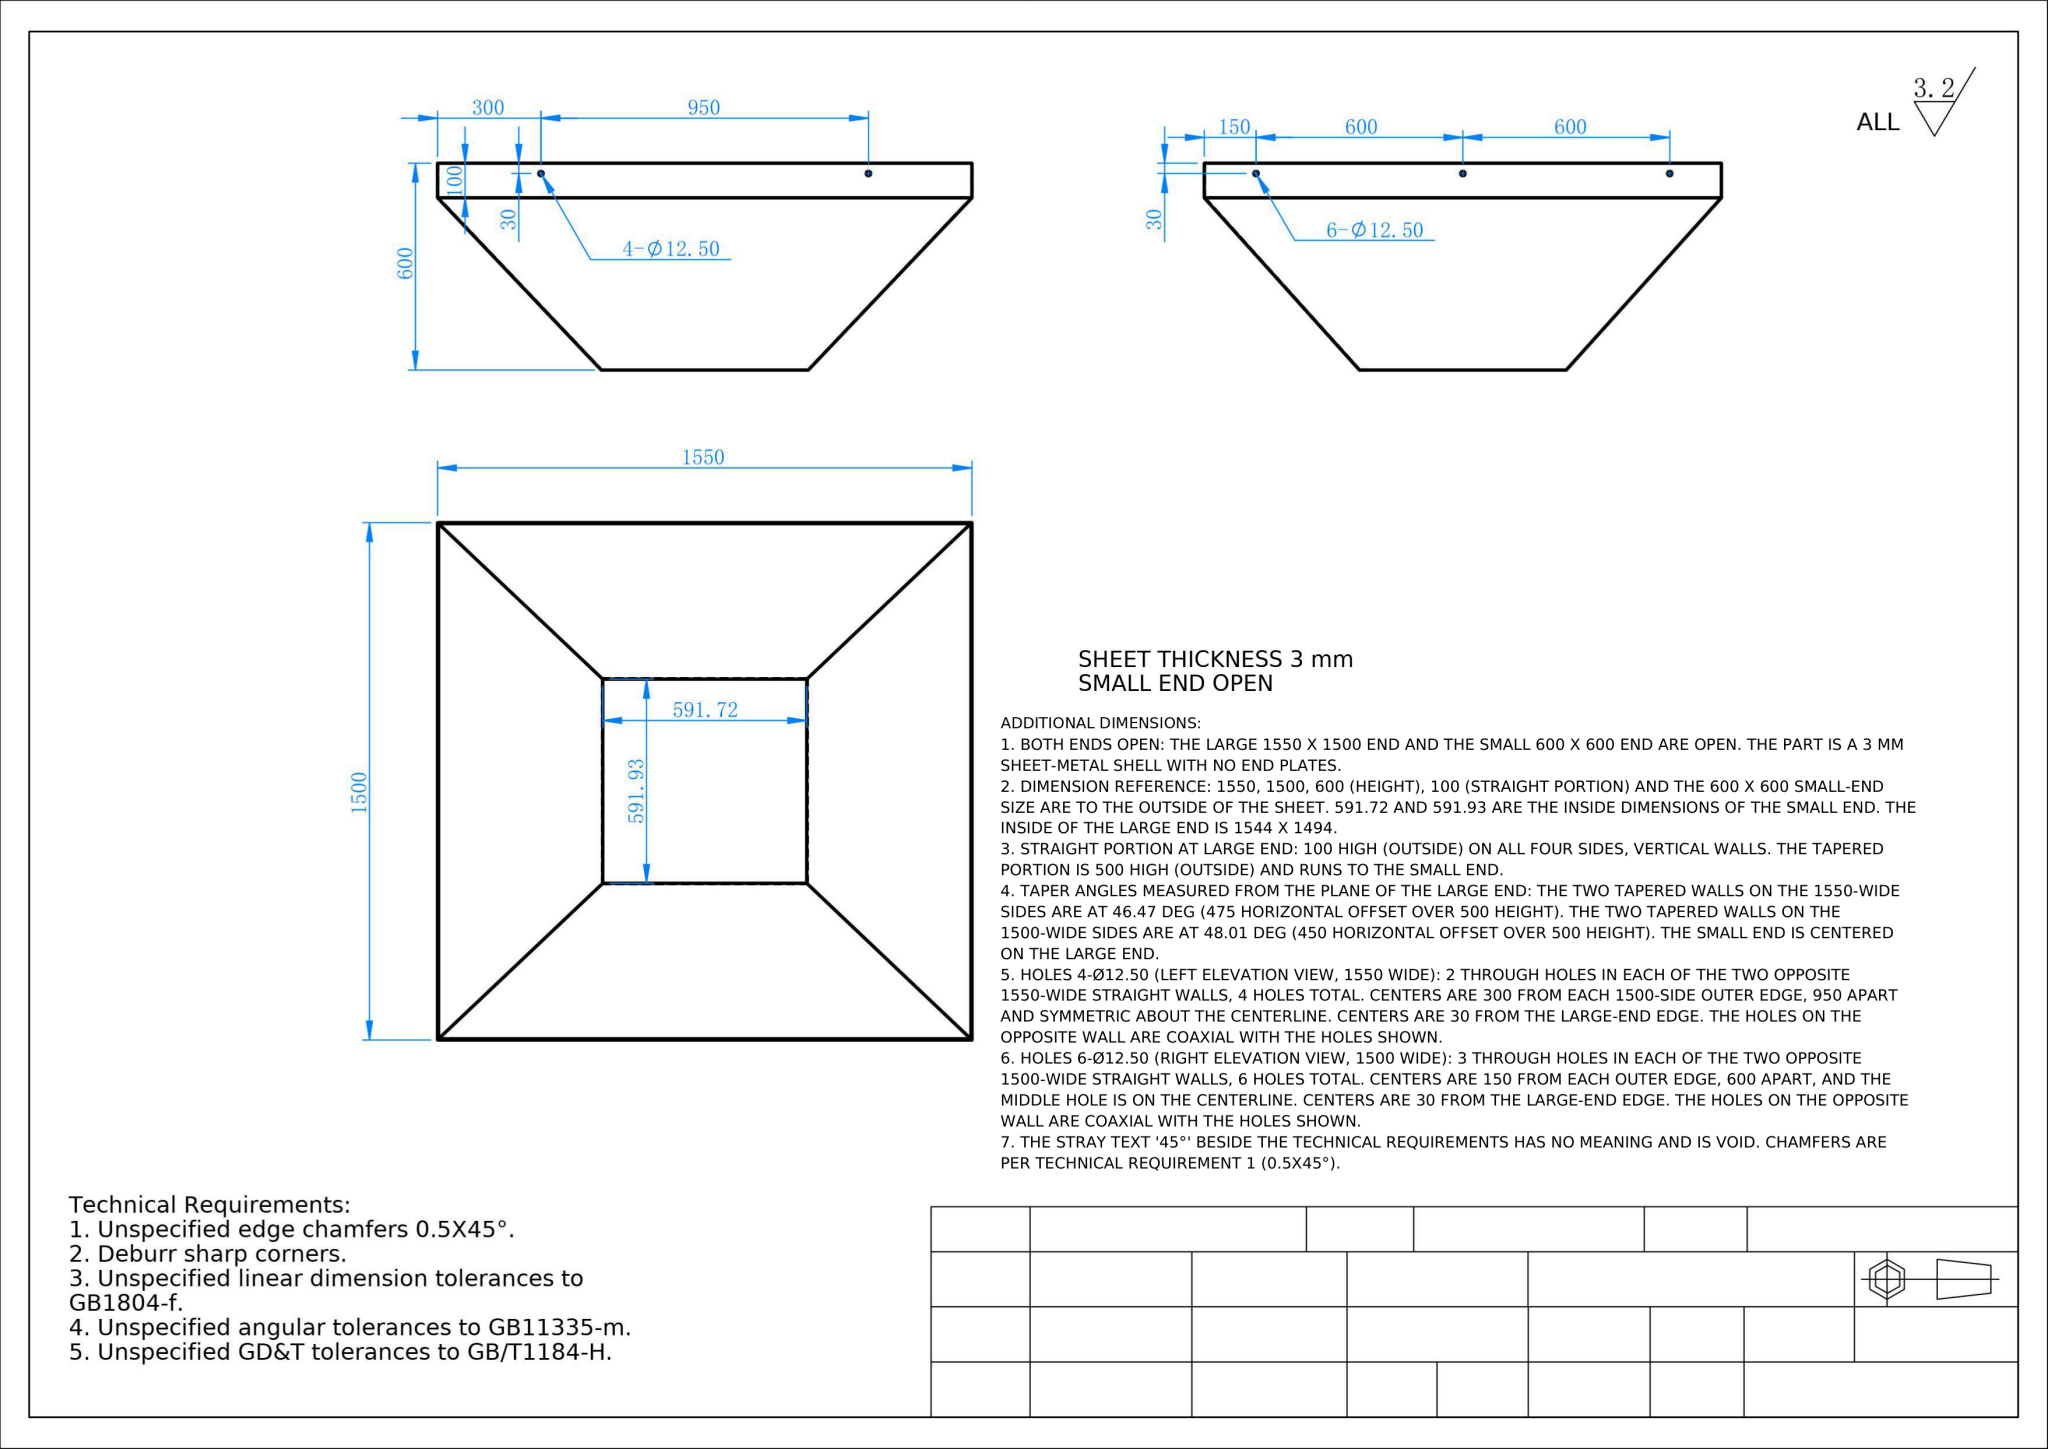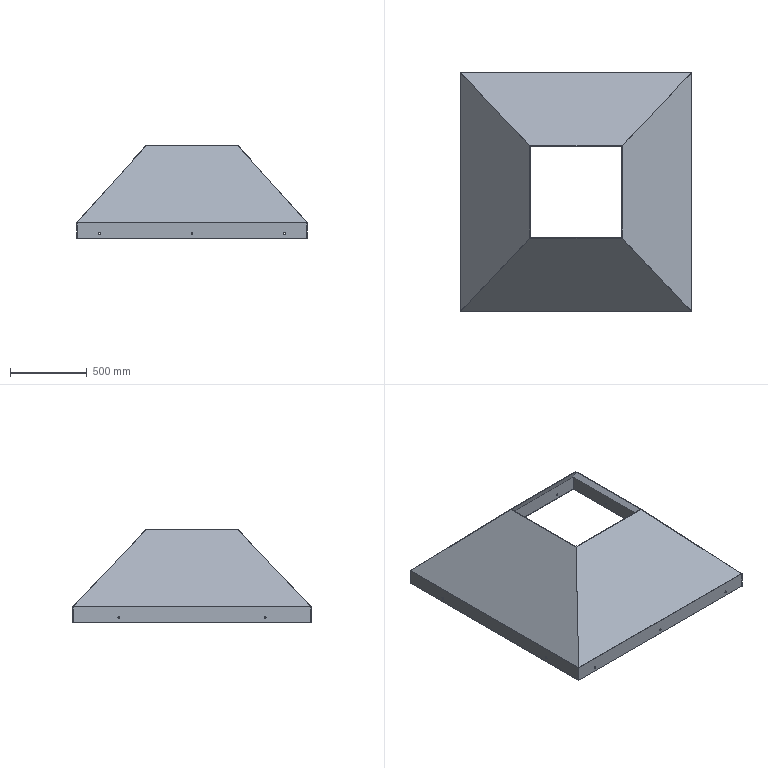Part | NX | mm | Diamond Aperture Mounting Plate | 1 solid | 38 faces | box 1500 x 1550 x 600 mm | volume 10476817 mm3 | cylinder 20 | plane 18 | commonest cylinder face diameters 12.5 x20